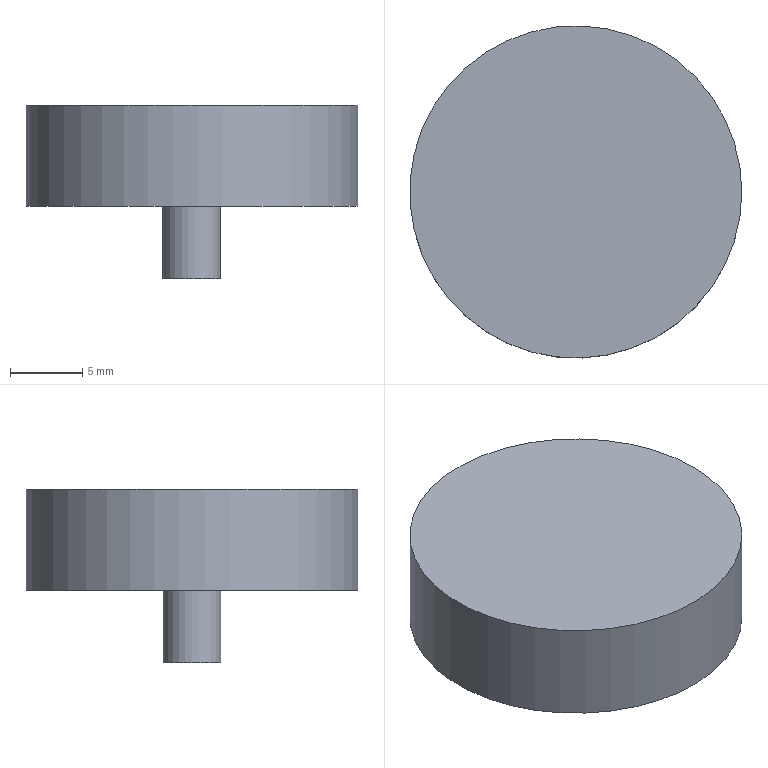Component | NX | MOTOR_DIAGRAM | 1 solid | 5 faces | box 23 x 23 x 12 mm | volume 2971 mm3 | plane 3 | cylinder 2 | commonest cylinder face diameters 23 x1 4 x1
STEP:
#1=CARTESIAN_POINT('',(0.,0.,0.));
#2=DIRECTION('',(0.,0.,1.));
#3=DIRECTION('',(1.,0.,0.));
#4=AXIS2_PLACEMENT_3D('',#1,#2,#3);
#5=CARTESIAN_POINT('',(11.5,-19.,14.));
#6=VERTEX_POINT('',#5);
#7=CARTESIAN_POINT('',(-0.,-19.,14.));
#8=DIRECTION('',(0.,0.,1.));
#9=DIRECTION('',(1.,0.,0.));
#10=AXIS2_PLACEMENT_3D('',#7,#8,#9);
#11=CIRCLE('',#10,11.5);
#12=CARTESIAN_POINT('',(-0.,-19.,14.));
#13=DIRECTION('',(0.,0.,-1.));
#14=DIRECTION('',(-1.,0.,0.));
#15=AXIS2_PLACEMENT_3D('',#12,#13,#14);
#16=CYLINDRICAL_SURFACE('',#15,11.5);
#17=CARTESIAN_POINT('',(9.425,0.));
#18=DIRECTION('',(-1.,0.));
#19=VECTOR('',#18,1.);
#20=LINE('',#17,#19);
#21=(GEOMETRIC_REPRESENTATION_CONTEXT(2)PARAMETRIC_REPRESENTATION_CONTEXT()REPRESENTATION_CONTEXT('',''));
#22=DEFINITIONAL_REPRESENTATION('',(#20),#21);
#23=PCURVE('',#16,#22);
#24=CARTESIAN_POINT('',(-0.,-19.,14.));
#25=DIRECTION('',(0.,0.,1.));
#26=DIRECTION('',(1.,0.,0.));
#27=AXIS2_PLACEMENT_3D('',#24,#25,#26);
#28=PLANE('',#27);
#29=CARTESIAN_POINT('',(0.,0.));
#30=DIRECTION('',(1.,0.));
#31=AXIS2_PLACEMENT_2D('',#29,#30);
#32=CIRCLE('',#31,11.5);
#33=(GEOMETRIC_REPRESENTATION_CONTEXT(2)PARAMETRIC_REPRESENTATION_CONTEXT()REPRESENTATION_CONTEXT('',''));
#34=DEFINITIONAL_REPRESENTATION('',(#32),#33);
#35=PCURVE('',#28,#34);
#36=SURFACE_CURVE('',#11,(#23,#35),.PCURVE_S1.);
#37=EDGE_CURVE('',#6,#6,#36,.T.);
#38=ORIENTED_EDGE('',*,*,#37,.F.);
#39=CARTESIAN_POINT('',(11.5,-19.,7.));
#40=VERTEX_POINT('',#39);
#41=CARTESIAN_POINT('',(11.5,-19.,14.));
#42=CARTESIAN_POINT('',(11.5,-19.,7.));
#43=B_SPLINE_CURVE_WITH_KNOTS('',1,(#41,#42),.UNSPECIFIED.,.F.,.F.,(2,2),(0.,7.),.PIECEWISE_BEZIER_KNOTS.);
#44=CARTESIAN_POINT('',(9.425,0.));
#45=DIRECTION('',(0.,1.));
#46=VECTOR('',#45,1.);
#47=LINE('',#44,#46);
#48=(GEOMETRIC_REPRESENTATION_CONTEXT(2)PARAMETRIC_REPRESENTATION_CONTEXT()REPRESENTATION_CONTEXT('',''));
#49=DEFINITIONAL_REPRESENTATION('',(#47),#48);
#50=PCURVE('',#16,#49);
#51=CARTESIAN_POINT('',(3.142,0.));
#52=DIRECTION('',(0.,1.));
#53=VECTOR('',#52,1.);
#54=LINE('',#51,#53);
#55=(GEOMETRIC_REPRESENTATION_CONTEXT(2)PARAMETRIC_REPRESENTATION_CONTEXT()REPRESENTATION_CONTEXT('',''));
#56=DEFINITIONAL_REPRESENTATION('',(#54),#55);
#57=PCURVE('',#16,#56);
#58=SEAM_CURVE('',#43,(#50,#57),.PCURVE_S1.);
#59=EDGE_CURVE('',#6,#40,#58,.T.);
#60=ORIENTED_EDGE('',*,*,#59,.T.);
#61=CARTESIAN_POINT('',(-0.,-19.,7.));
#62=DIRECTION('',(0.,0.,1.));
#63=DIRECTION('',(1.,0.,0.));
#64=AXIS2_PLACEMENT_3D('',#61,#62,#63);
#65=CIRCLE('',#64,11.5);
#66=CARTESIAN_POINT('',(9.425,7.));
#67=DIRECTION('',(-1.,0.));
#68=VECTOR('',#67,1.);
#69=LINE('',#66,#68);
#70=(GEOMETRIC_REPRESENTATION_CONTEXT(2)PARAMETRIC_REPRESENTATION_CONTEXT()REPRESENTATION_CONTEXT('',''));
#71=DEFINITIONAL_REPRESENTATION('',(#69),#70);
#72=PCURVE('',#16,#71);
#73=CARTESIAN_POINT('',(-0.,-19.,7.));
#74=DIRECTION('',(0.,0.,1.));
#75=DIRECTION('',(1.,0.,0.));
#76=AXIS2_PLACEMENT_3D('',#73,#74,#75);
#77=PLANE('',#76);
#78=CARTESIAN_POINT('',(0.,0.));
#79=DIRECTION('',(1.,0.));
#80=AXIS2_PLACEMENT_2D('',#78,#79);
#81=CIRCLE('',#80,11.5);
#82=(GEOMETRIC_REPRESENTATION_CONTEXT(2)PARAMETRIC_REPRESENTATION_CONTEXT()REPRESENTATION_CONTEXT('',''));
#83=DEFINITIONAL_REPRESENTATION('',(#81),#82);
#84=PCURVE('',#77,#83);
#85=SURFACE_CURVE('',#65,(#72,#84),.PCURVE_S1.);
#86=EDGE_CURVE('',#40,#40,#85,.T.);
#87=ORIENTED_EDGE('',*,*,#86,.T.);
#88=ORIENTED_EDGE('',*,*,#59,.F.);
#89=EDGE_LOOP('',(#38,#60,#87,#88));
#90=FACE_BOUND('',#89,.T.);
#91=ADVANCED_FACE('',(#90),#16,.T.);
#92=ORIENTED_EDGE('',*,*,#37,.T.);
#93=EDGE_LOOP('',(#92));
#94=FACE_BOUND('',#93,.T.);
#95=ADVANCED_FACE('',(#94),#28,.T.);
#96=CARTESIAN_POINT('',(2.,-19.,7.));
#97=VERTEX_POINT('',#96);
#98=CARTESIAN_POINT('',(-0.,-19.,7.));
#99=DIRECTION('',(0.,0.,-1.));
#100=DIRECTION('',(1.,0.,0.));
#101=AXIS2_PLACEMENT_3D('',#98,#99,#100);
#102=CIRCLE('',#101,2.);
#103=CARTESIAN_POINT('',(2.,0.));
#104=CARTESIAN_POINT('',(2.,-3.464));
#105=CARTESIAN_POINT('',(-1.,-1.732));
#106=CARTESIAN_POINT('',(-4.,-0.));
#107=CARTESIAN_POINT('',(-1.,1.732));
#108=CARTESIAN_POINT('',(2.,3.464));
#109=CARTESIAN_POINT('',(2.,0.));
#110=(BOUNDED_CURVE()B_SPLINE_CURVE(2,(#103,#104,#105,#106,#107,#108,#109),.UNSPECIFIED.,.T.,.F.)B_SPLINE_CURVE_WITH_KNOTS((1,2,2,2,2,1),(-2.094,0.,2.094,4.189,6.283,8.378),.UNSPECIFIED.)CURVE()GEOMETRIC_REPRESENTATION_ITEM()RATIONAL_B_SPLINE_CURVE((1.,0.5,1.,0.5,1.,0.5,1.))REPRESENTATION_ITEM(''));
#111=(GEOMETRIC_REPRESENTATION_CONTEXT(2)PARAMETRIC_REPRESENTATION_CONTEXT()REPRESENTATION_CONTEXT('',''));
#112=DEFINITIONAL_REPRESENTATION('',(#110),#111);
#113=PCURVE('',#77,#112);
#114=CARTESIAN_POINT('',(-0.,-19.,2.));
#115=DIRECTION('',(0.,0.,1.));
#116=DIRECTION('',(1.,0.,0.));
#117=AXIS2_PLACEMENT_3D('',#114,#115,#116);
#118=CYLINDRICAL_SURFACE('',#117,2.);
#119=CARTESIAN_POINT('',(6.283,5.));
#120=DIRECTION('',(-1.,0.));
#121=VECTOR('',#120,1.);
#122=LINE('',#119,#121);
#123=(GEOMETRIC_REPRESENTATION_CONTEXT(2)PARAMETRIC_REPRESENTATION_CONTEXT()REPRESENTATION_CONTEXT('',''));
#124=DEFINITIONAL_REPRESENTATION('',(#122),#123);
#125=PCURVE('',#118,#124);
#126=SURFACE_CURVE('',#102,(#113,#125),.PCURVE_S1.);
#127=EDGE_CURVE('',#97,#97,#126,.T.);
#128=ORIENTED_EDGE('',*,*,#127,.F.);
#129=EDGE_LOOP('',(#128));
#130=FACE_BOUND('',#129,.T.);
#131=ORIENTED_EDGE('',*,*,#86,.F.);
#132=EDGE_LOOP('',(#131));
#133=FACE_BOUND('',#132,.T.);
#134=ADVANCED_FACE('',(#130,#133),#77,.F.);
#135=CARTESIAN_POINT('',(2.,-19.,2.));
#136=VERTEX_POINT('',#135);
#137=CARTESIAN_POINT('',(-0.,-19.,2.));
#138=DIRECTION('',(0.,0.,-1.));
#139=DIRECTION('',(1.,0.,0.));
#140=AXIS2_PLACEMENT_3D('',#137,#138,#139);
#141=CIRCLE('',#140,2.);
#142=CARTESIAN_POINT('',(6.283,0.));
#143=DIRECTION('',(-1.,0.));
#144=VECTOR('',#143,1.);
#145=LINE('',#142,#144);
#146=(GEOMETRIC_REPRESENTATION_CONTEXT(2)PARAMETRIC_REPRESENTATION_CONTEXT()REPRESENTATION_CONTEXT('',''));
#147=DEFINITIONAL_REPRESENTATION('',(#145),#146);
#148=PCURVE('',#118,#147);
#149=CARTESIAN_POINT('',(-0.,-19.,2.));
#150=DIRECTION('',(0.,0.,-1.));
#151=DIRECTION('',(-1.,0.,0.));
#152=AXIS2_PLACEMENT_3D('',#149,#150,#151);
#153=PLANE('',#152);
#154=CARTESIAN_POINT('',(0.,0.));
#155=DIRECTION('',(-1.,0.));
#156=AXIS2_PLACEMENT_2D('',#154,#155);
#157=CIRCLE('',#156,2.);
#158=(GEOMETRIC_REPRESENTATION_CONTEXT(2)PARAMETRIC_REPRESENTATION_CONTEXT()REPRESENTATION_CONTEXT('',''));
#159=DEFINITIONAL_REPRESENTATION('',(#157),#158);
#160=PCURVE('',#153,#159);
#161=SURFACE_CURVE('',#141,(#148,#160),.PCURVE_S1.);
#162=EDGE_CURVE('',#136,#136,#161,.T.);
#163=ORIENTED_EDGE('',*,*,#162,.F.);
#164=CARTESIAN_POINT('',(2.,-19.,2.));
#165=CARTESIAN_POINT('',(2.,-19.,7.));
#166=B_SPLINE_CURVE_WITH_KNOTS('',1,(#164,#165),.UNSPECIFIED.,.F.,.F.,(2,2),(0.,5.),.PIECEWISE_BEZIER_KNOTS.);
#167=CARTESIAN_POINT('',(6.283,0.));
#168=DIRECTION('',(0.,1.));
#169=VECTOR('',#168,1.);
#170=LINE('',#167,#169);
#171=(GEOMETRIC_REPRESENTATION_CONTEXT(2)PARAMETRIC_REPRESENTATION_CONTEXT()REPRESENTATION_CONTEXT('',''));
#172=DEFINITIONAL_REPRESENTATION('',(#170),#171);
#173=PCURVE('',#118,#172);
#174=CARTESIAN_POINT('',(0.,0.));
#175=DIRECTION('',(0.,1.));
#176=VECTOR('',#175,1.);
#177=LINE('',#174,#176);
#178=(GEOMETRIC_REPRESENTATION_CONTEXT(2)PARAMETRIC_REPRESENTATION_CONTEXT()REPRESENTATION_CONTEXT('',''));
#179=DEFINITIONAL_REPRESENTATION('',(#177),#178);
#180=PCURVE('',#118,#179);
#181=SEAM_CURVE('',#166,(#173,#180),.PCURVE_S1.);
#182=EDGE_CURVE('',#136,#97,#181,.T.);
#183=ORIENTED_EDGE('',*,*,#182,.T.);
#184=ORIENTED_EDGE('',*,*,#127,.T.);
#185=ORIENTED_EDGE('',*,*,#182,.F.);
#186=EDGE_LOOP('',(#163,#183,#184,#185));
#187=FACE_BOUND('',#186,.T.);
#188=ADVANCED_FACE('',(#187),#118,.T.);
#189=ORIENTED_EDGE('',*,*,#162,.T.);
#190=EDGE_LOOP('',(#189));
#191=FACE_BOUND('',#190,.T.);
#192=ADVANCED_FACE('',(#191),#153,.T.);
#193=CLOSED_SHELL('',(#91,#95,#134,#188,#192));
#194=MANIFOLD_SOLID_BREP('',#193);
#195=(LENGTH_UNIT()NAMED_UNIT(*)SI_UNIT(.MILLI.,.METRE.));
#196=UNCERTAINTY_MEASURE_WITH_UNIT(LENGTH_MEASURE(0.00001),#195,'','');
#197=(NAMED_UNIT(*)PLANE_ANGLE_UNIT()SI_UNIT($,.RADIAN.));
#198=(NAMED_UNIT(*)SI_UNIT($,.STERADIAN.)SOLID_ANGLE_UNIT());
#199=(GEOMETRIC_REPRESENTATION_CONTEXT(3)GLOBAL_UNCERTAINTY_ASSIGNED_CONTEXT((#196))GLOBAL_UNIT_ASSIGNED_CONTEXT((#195,#197,#198))REPRESENTATION_CONTEXT('',''));
#200=ADVANCED_BREP_SHAPE_REPRESENTATION('',(#4,#194),#199);